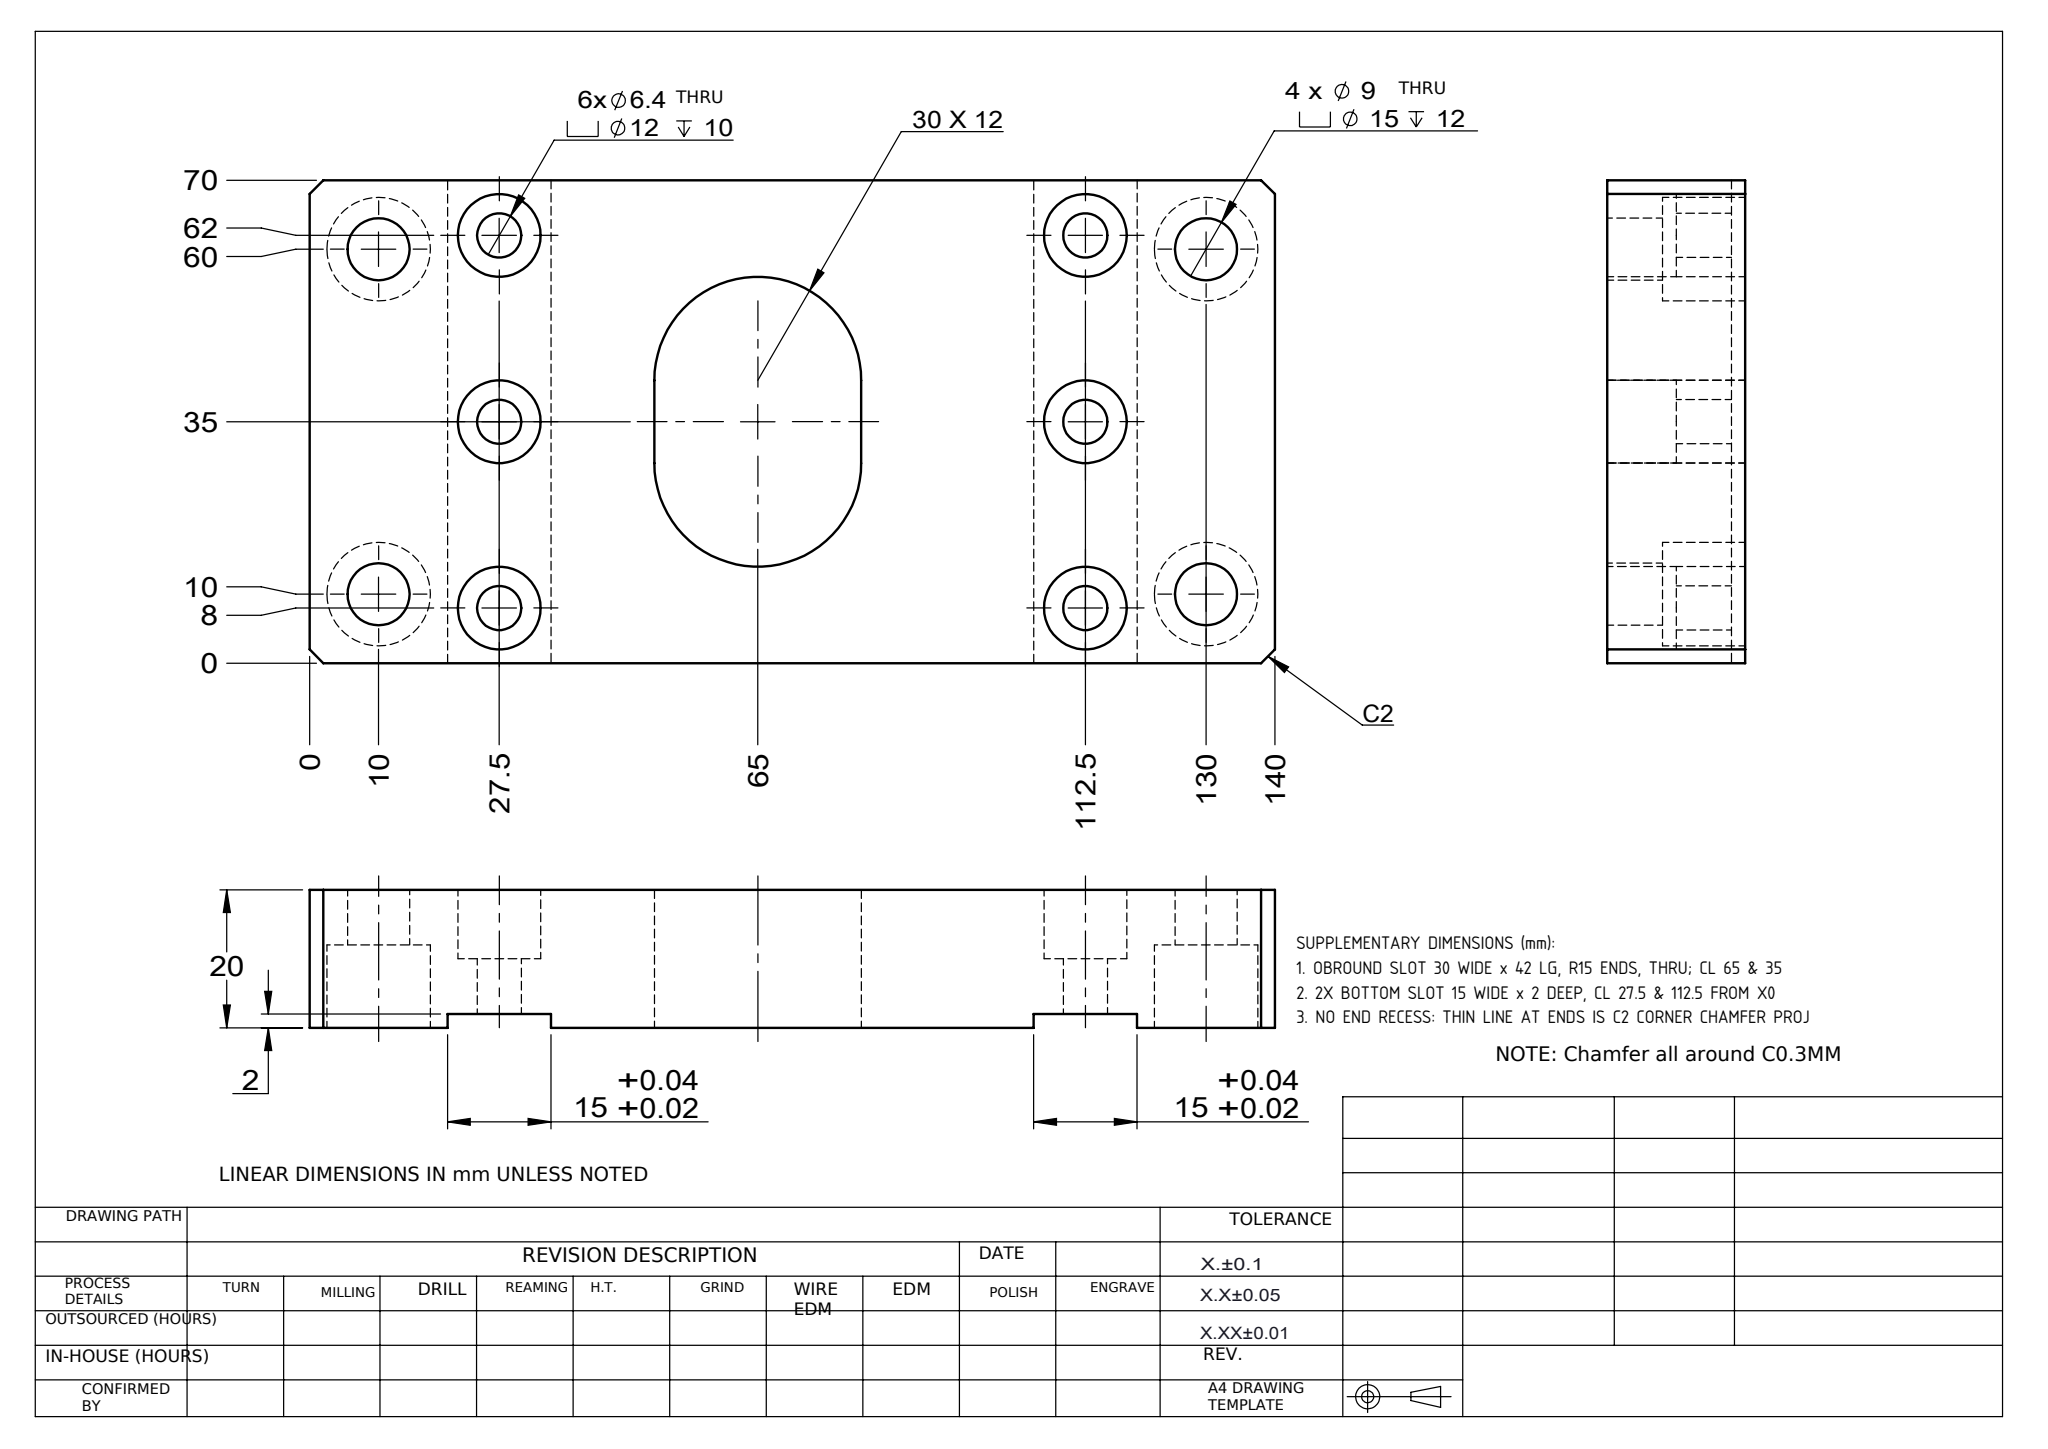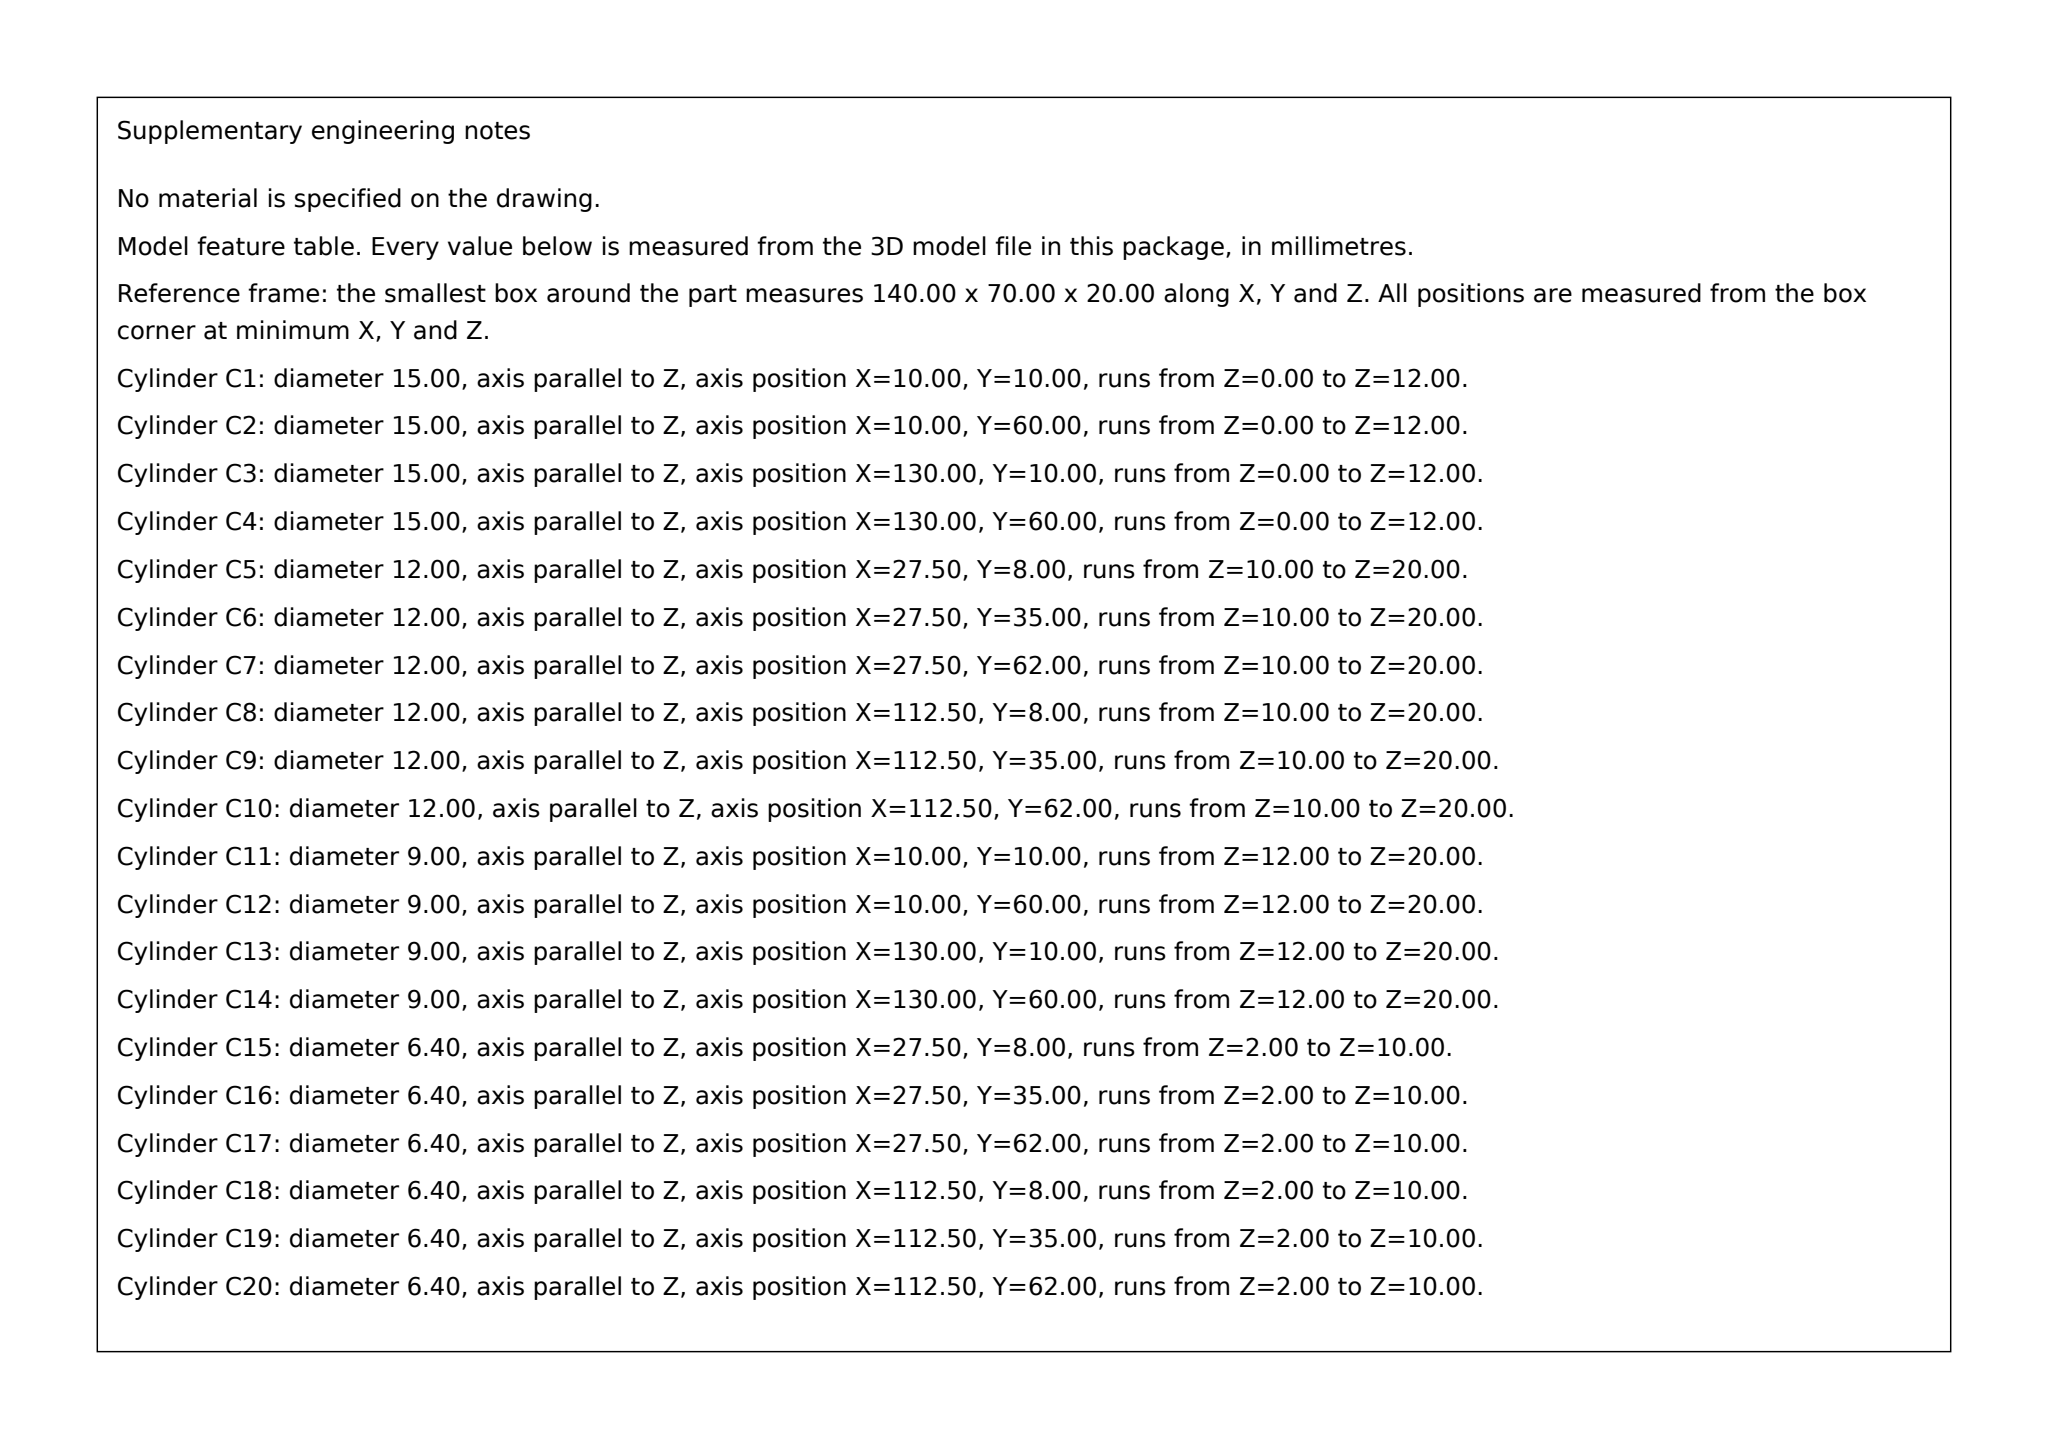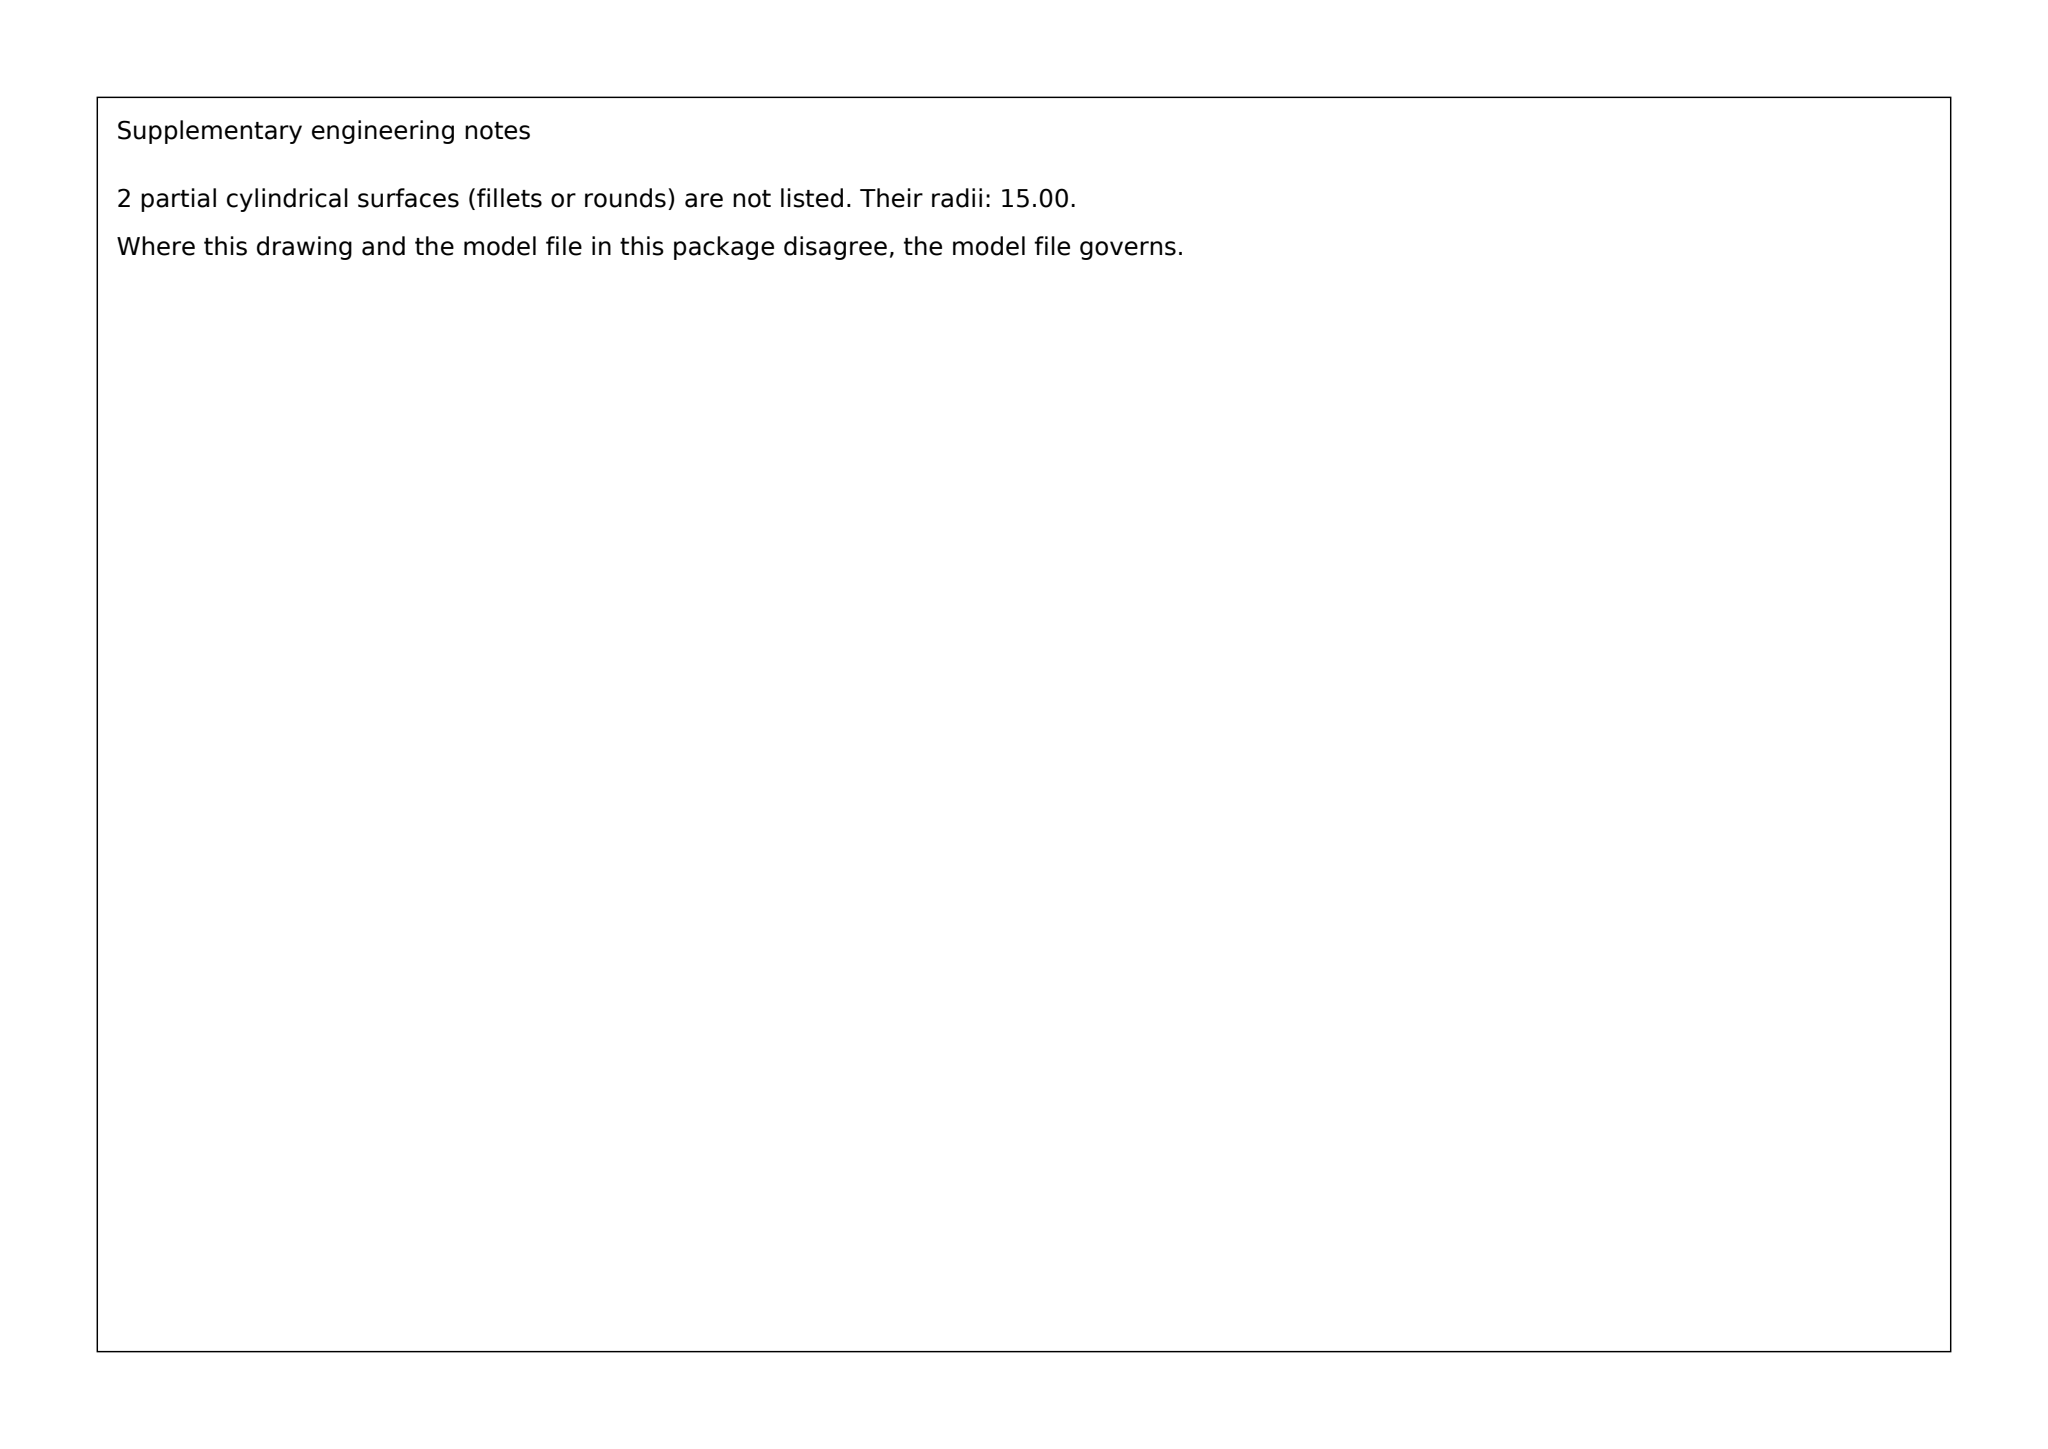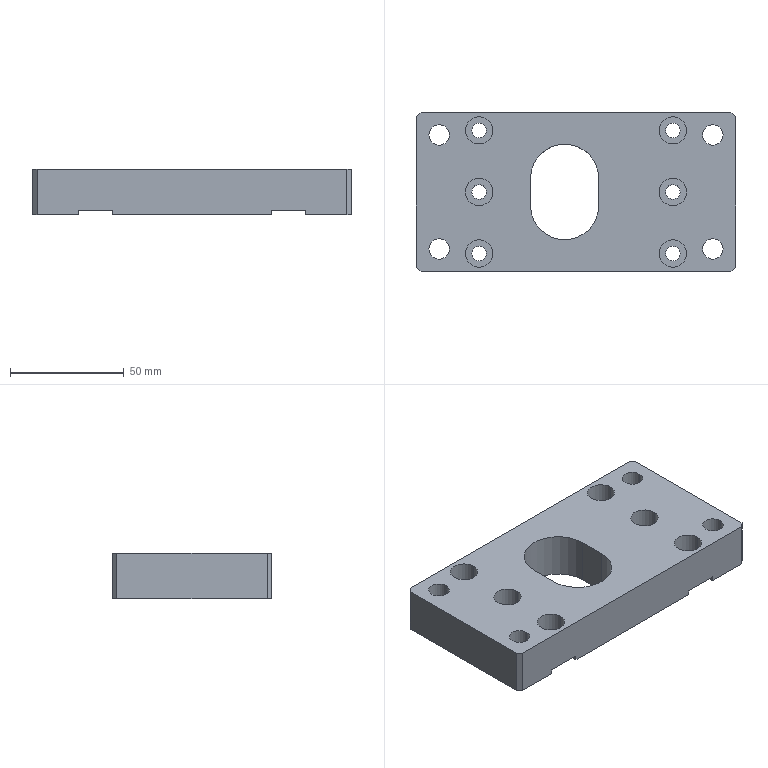Part | SolidWorks | mm | 1 solid | 72 faces | box 140 x 70 x 20 mm | volume 151455 mm3 | cylinder 42 | plane 30 | commonest cylinder face diameters 12 x12 6.4 x12 15 x8 9 x8 30 x2
build123d program:
from build123d import *

# Parameters (mm, degrees)
SKETCH1_W                                       = 140
SKETCH1_H                                       = 70
BOSS_EXTRUDE1_DEPTH                             = 20
M8_HEX_SOCKET_HEAD_CAP_SCREW_CBORE1_D           = 9
M8_HEX_SOCKET_HEAD_CAP_SCREW_CBORE1_CBORE_D     = 15
M8_HEX_SOCKET_HEAD_CAP_SCREW_CBORE1_CBORE_DEPTH = 12
CHAMFER1_SIZE                                   = 2
SKETCH9_W                                       = 15
SKETCH9_H                                       = 111.091
SKETCH9_H_2                                     = 141.839
CUT_EXTRUDE6_DEPTH                              = 2
SKETCH10_R                                      = 3.2
CUT_EXTRUDE7_DEPTH                              = 158.556
SKETCH11_R                                      = 6
CUT_EXTRUDE8_DEPTH                              = 10
CUT_EXTRUDE9_DEPTH                              = 158.797
CUT_EXTRUDE9_DEPTH_BACK                         = 158.797


with BuildPart() as part:
    # Sketch1 → Boss-Extrude1 (new body)
    with BuildSketch(Plane.XY):
        with Locations((70, 35)):
            Rectangle(SKETCH1_W, SKETCH1_H)
    extrude(amount=BOSS_EXTRUDE1_DEPTH)

    # M8 Hex Socket Head Cap Screw CBORE1 (through all)
    with Locations(Plane(origin=(0, 0, 0), x_dir=(-1, 0, 0), z_dir=(0, 0, -1))):
        with Locations((-130, 60), (-130, 10), (-10, 60), (-10, 10)):
            CounterBoreHole(M8_HEX_SOCKET_HEAD_CAP_SCREW_CBORE1_D / 2, M8_HEX_SOCKET_HEAD_CAP_SCREW_CBORE1_CBORE_D / 2, M8_HEX_SOCKET_HEAD_CAP_SCREW_CBORE1_CBORE_DEPTH)

    # Chamfer1
    chamfer1_edges = [part.edges().sort_by_distance(p)[0] for p in [
        (0, 70, 10),
        (140, 70, 10),
        (140, 0, 10),
        (0, 0, 10),
    ]]
    chamfer(chamfer1_edges, length=CHAMFER1_SIZE)

    # Sketch9 → Cut-Extrude6 (cut)
    with BuildSketch(Plane(origin=(0, 0, 0), x_dir=(-1, 0, 0), z_dir=(0, 0, -1))):
        with Locations((-112.5, 39.794)):
            Rectangle(SKETCH9_W, SKETCH9_H)
        with Locations((-27.5, 35.331)):
            Rectangle(SKETCH9_W, SKETCH9_H_2)
    extrude(amount=-CUT_EXTRUDE6_DEPTH, mode=Mode.SUBTRACT)

    # Sketch10 → Cut-Extrude7 (cut, through all)
    with BuildSketch(Plane(origin=(0, 0, 2), x_dir=(-1, 0, 0), z_dir=(0, 0, -1))):
        with Locations((-112.5, 62)):
            Circle(SKETCH10_R)
        with Locations((-112.5, 35)):
            Circle(SKETCH10_R)
        with Locations((-112.5, 8)):
            Circle(SKETCH10_R)
        with Locations((-27.5, 62)):
            Circle(SKETCH10_R)
        with Locations((-27.5, 35)):
            Circle(SKETCH10_R)
        with Locations((-27.5, 8)):
            Circle(SKETCH10_R)
    extrude(amount=-CUT_EXTRUDE7_DEPTH, mode=Mode.SUBTRACT)

    # Sketch11 → Cut-Extrude8 (cut)
    with BuildSketch(Plane.XY.offset(20)):
        with Locations((27.5, 62)):
            Circle(SKETCH11_R)
        with Locations((27.5, 35)):
            Circle(SKETCH11_R)
        with Locations((27.5, 8)):
            Circle(SKETCH11_R)
        with Locations((112.5, 8)):
            Circle(SKETCH11_R)
        with Locations((112.5, 35)):
            Circle(SKETCH11_R)
        with Locations((112.5, 62)):
            Circle(SKETCH11_R)
    extrude(amount=-CUT_EXTRUDE8_DEPTH, mode=Mode.SUBTRACT)

    # Sketch12 → Cut-Extrude9 (cut, two sides: drawn at the far end of the back side and taken through both)
    with BuildSketch(Plane(origin=(0, 0, 0), x_dir=(-1, 0, 0), z_dir=(0, 0, -1)).offset(-CUT_EXTRUDE9_DEPTH_BACK)):
        with BuildLine():
            Line((-50, 41), (-50, 29))
            ThreePointArc((-50, 29), (-65, 14), (-80, 29))
            Line((-80, 29), (-80, 41))
            ThreePointArc((-80, 41), (-65, 56), (-50, 41))
        make_face()
    extrude(amount=CUT_EXTRUDE9_DEPTH + CUT_EXTRUDE9_DEPTH_BACK, mode=Mode.SUBTRACT)


solid = part.part